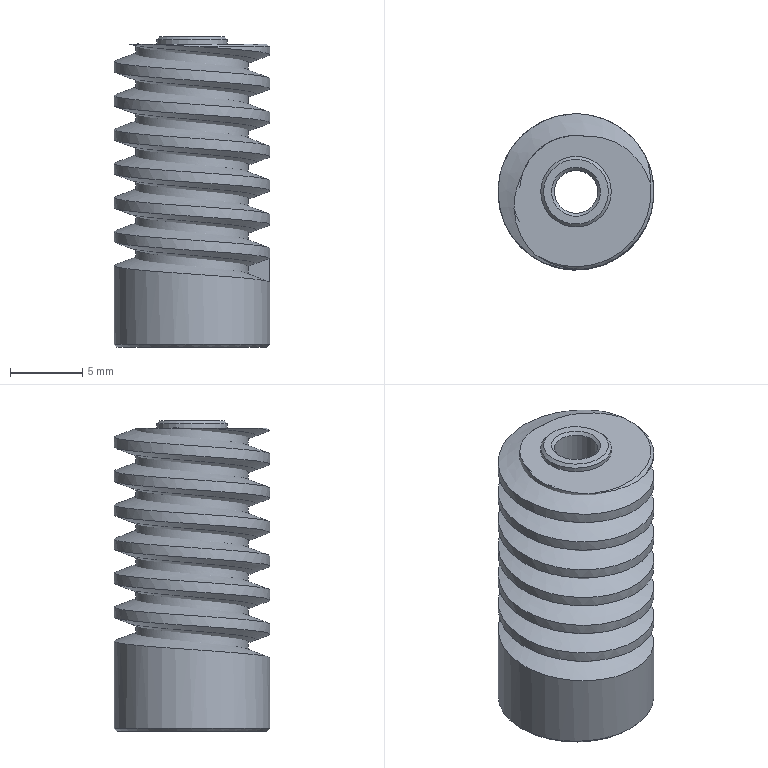Component | NX | DJZ_05_WORM_SHAFT_TRAVEL10 | 1 solid | 25 faces | volume 1360 mm3 | cylinder 11 | plane 6 | cone 6 | spline 2 | commonest cylinder face diameters 10.8 x8 5.2 x1 4.9 x1 3 x1